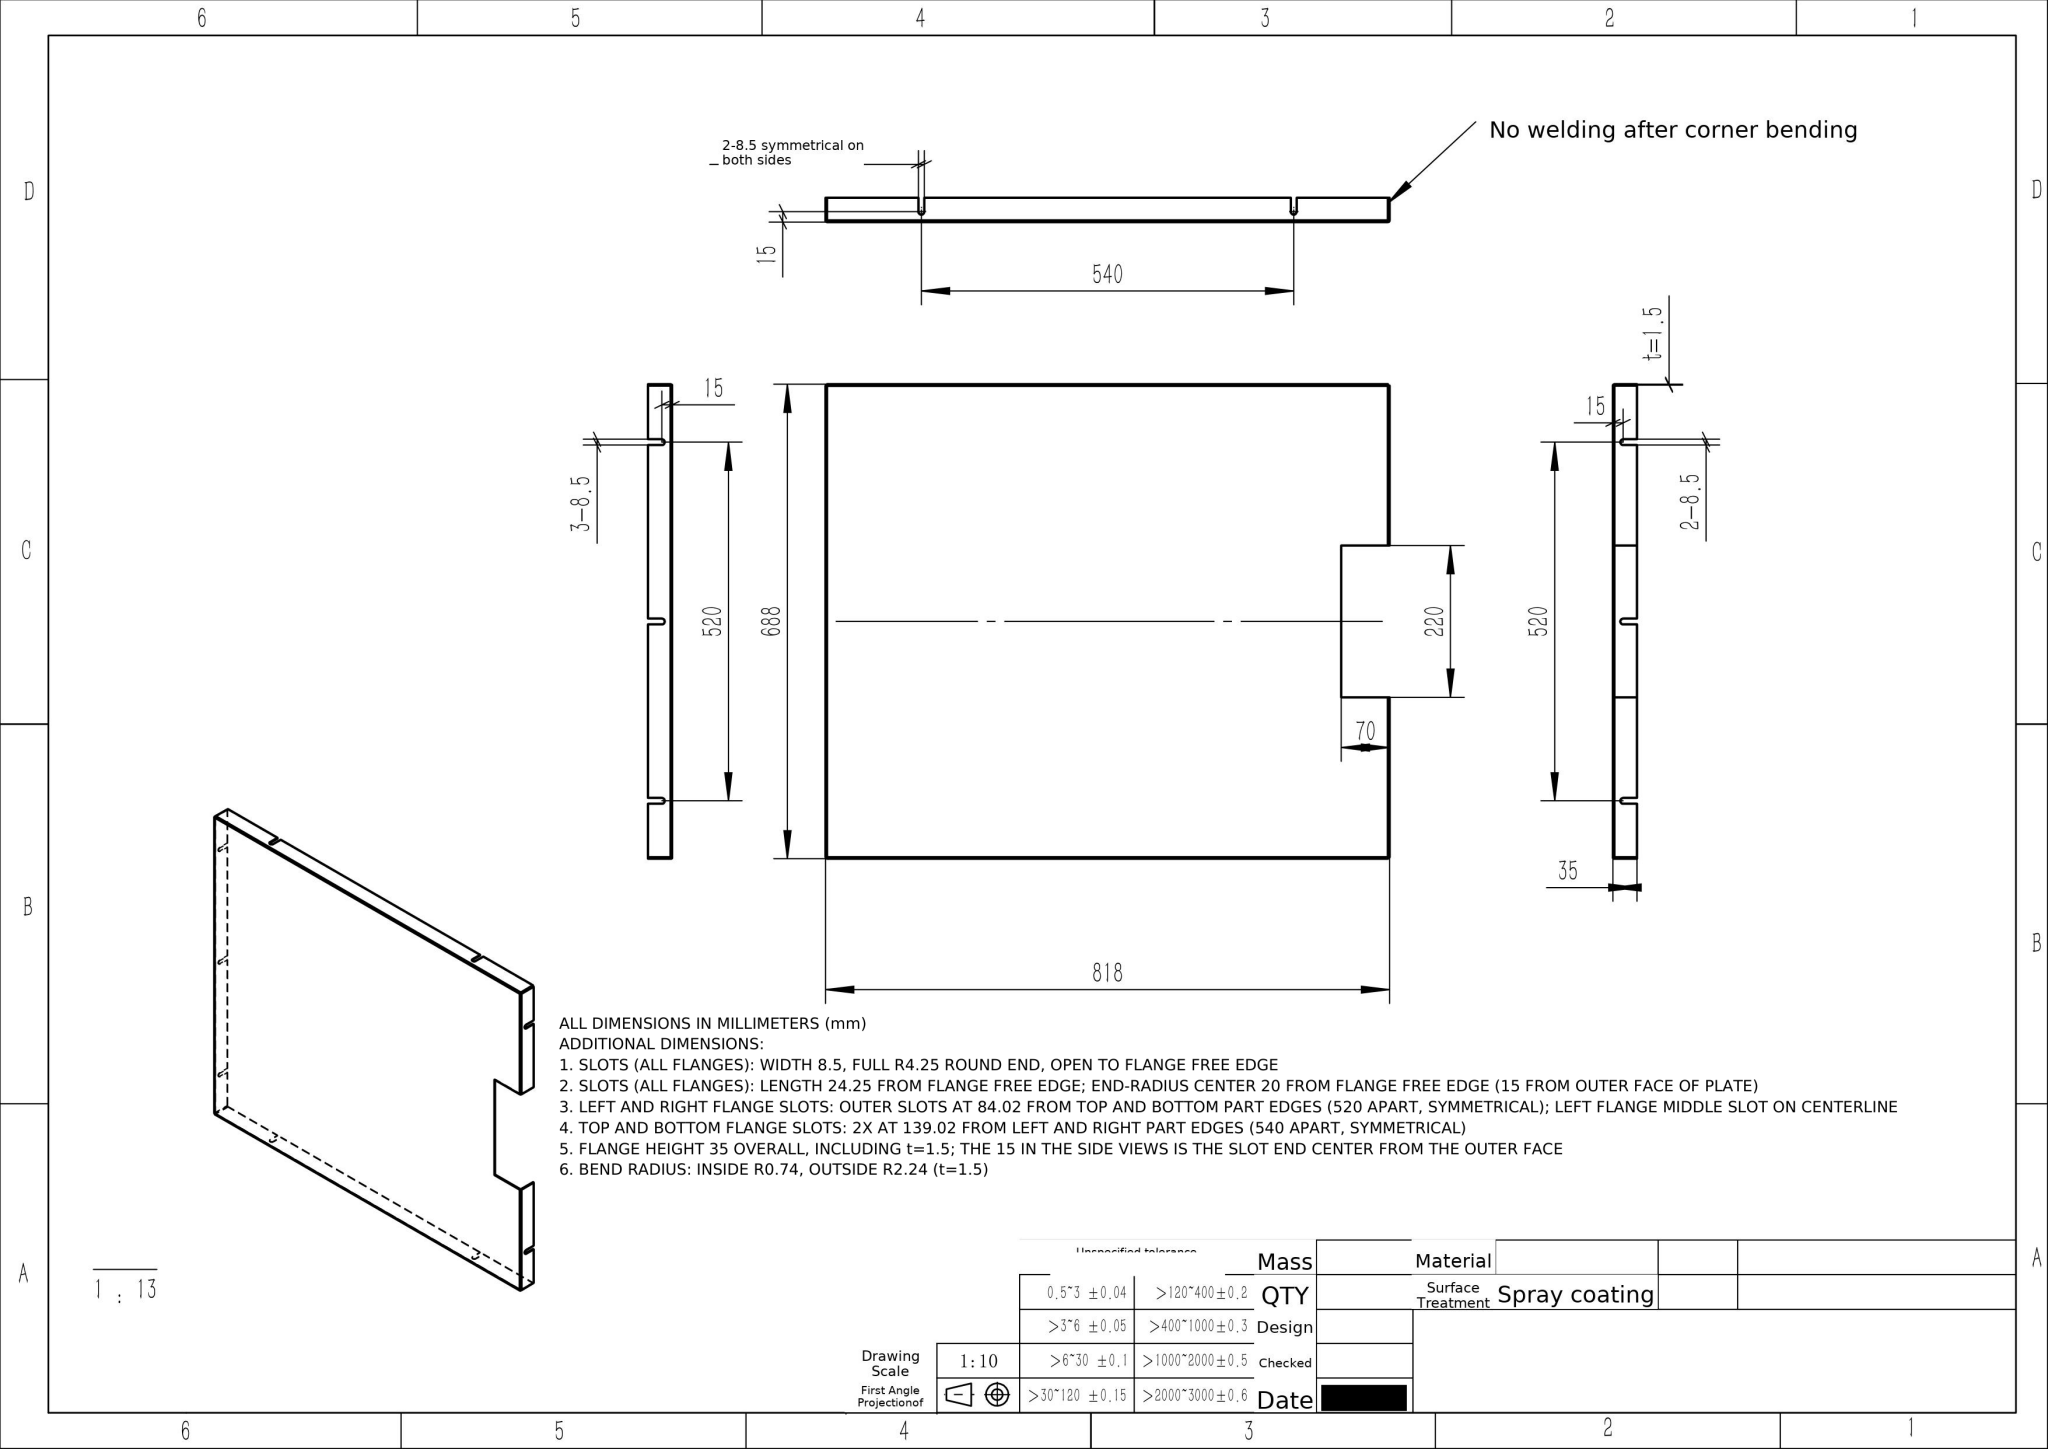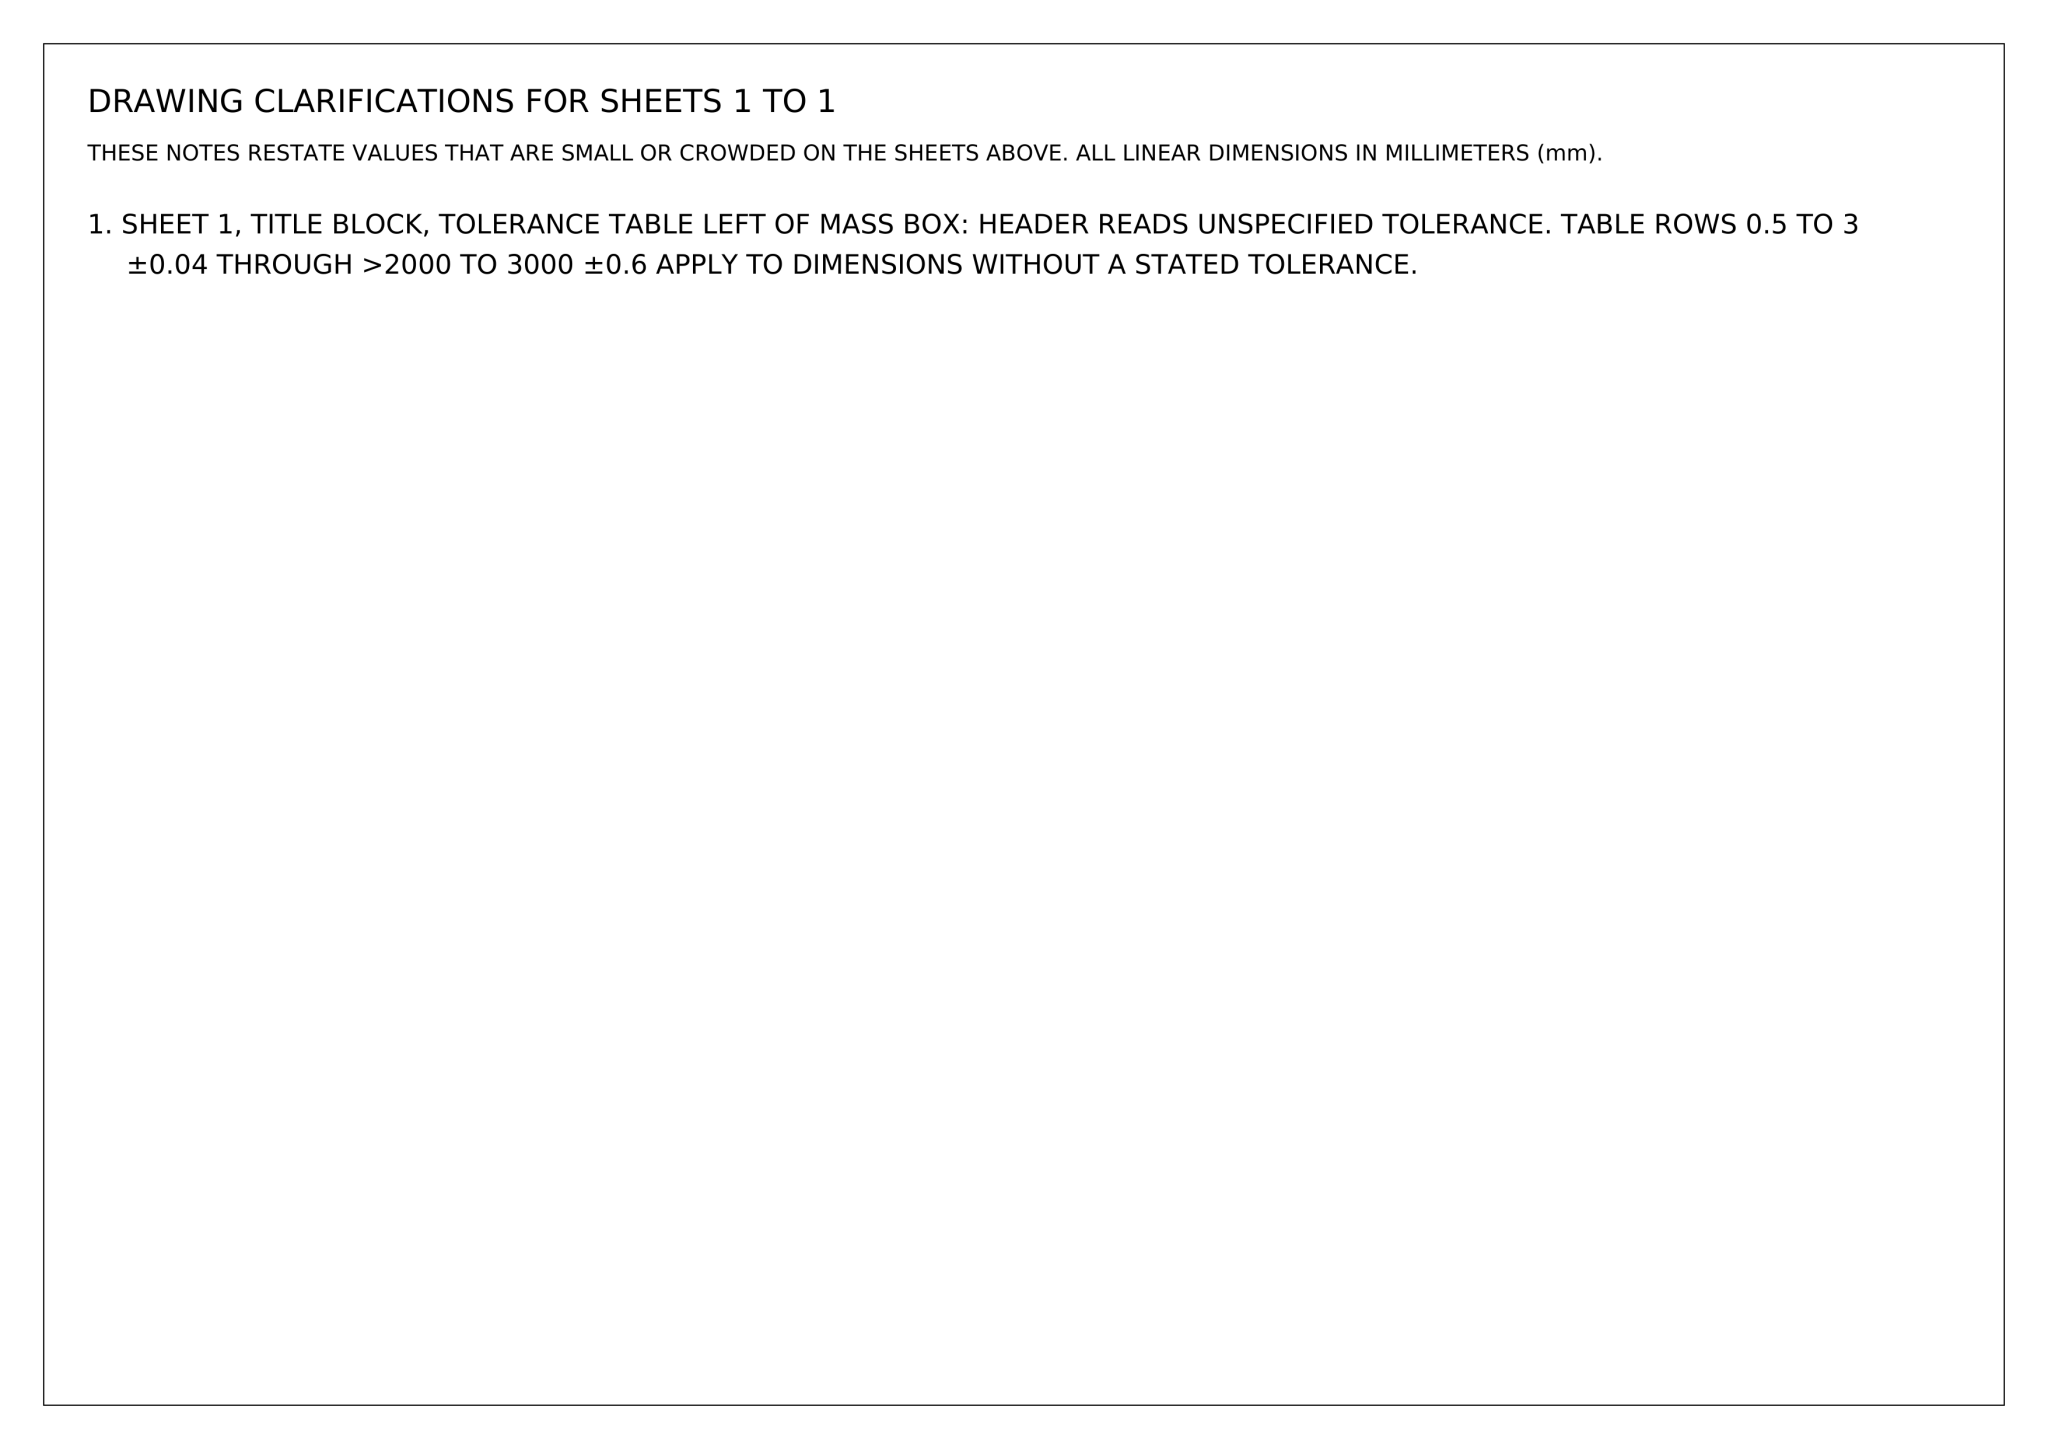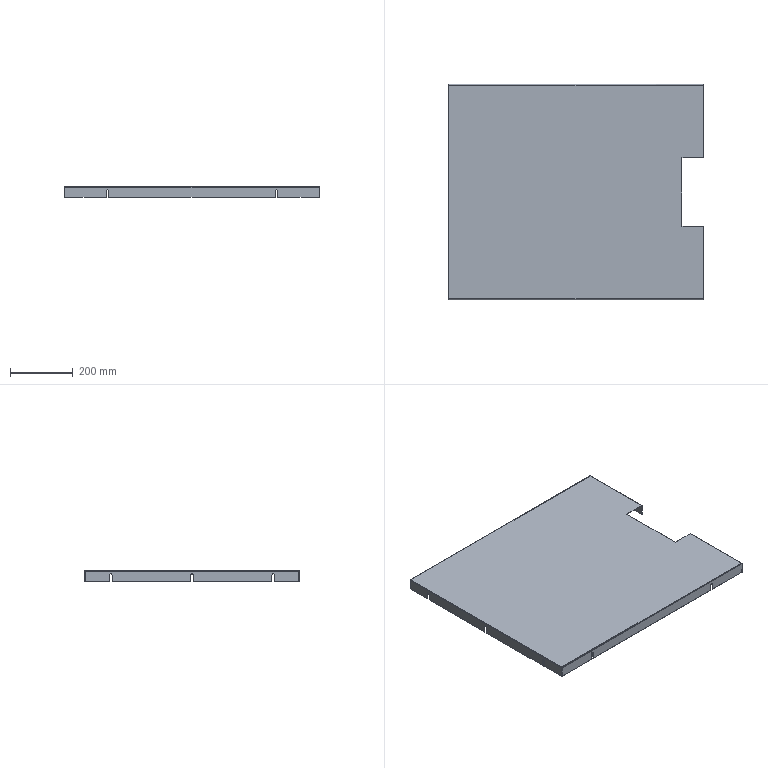Part | NX | mm | 1 solid | 90 faces | box 818 x 688 x 35 mm | volume 955124 mm3 | plane 59 | cylinder 23 | spline 8 | commonest cylinder face diameters 8.5 x13 4.473 x5 1.473 x5